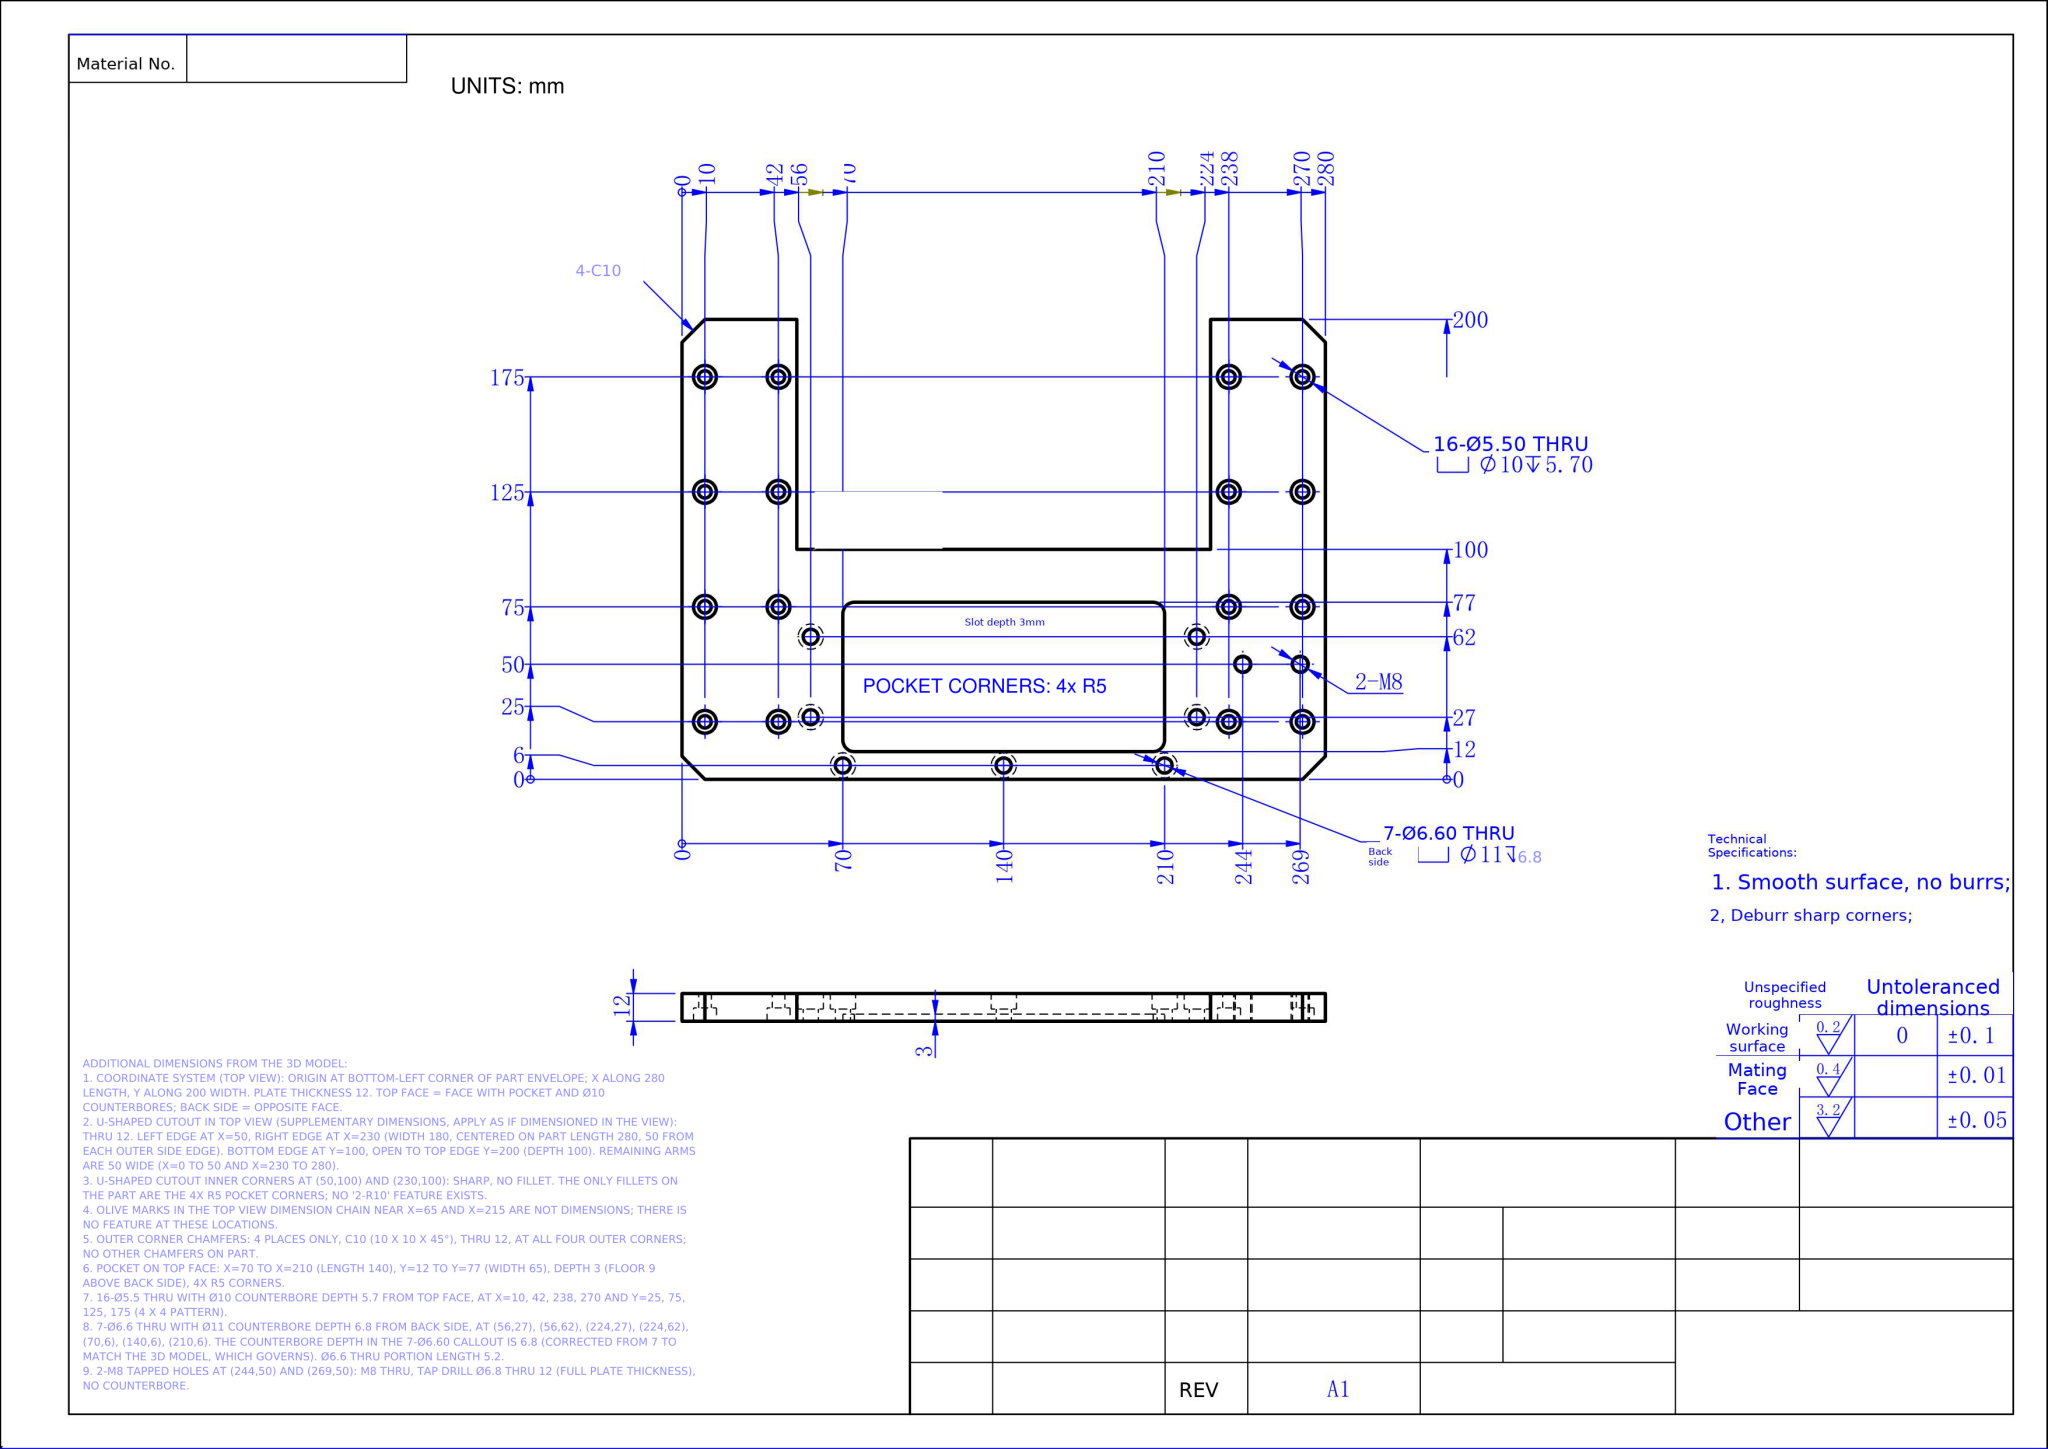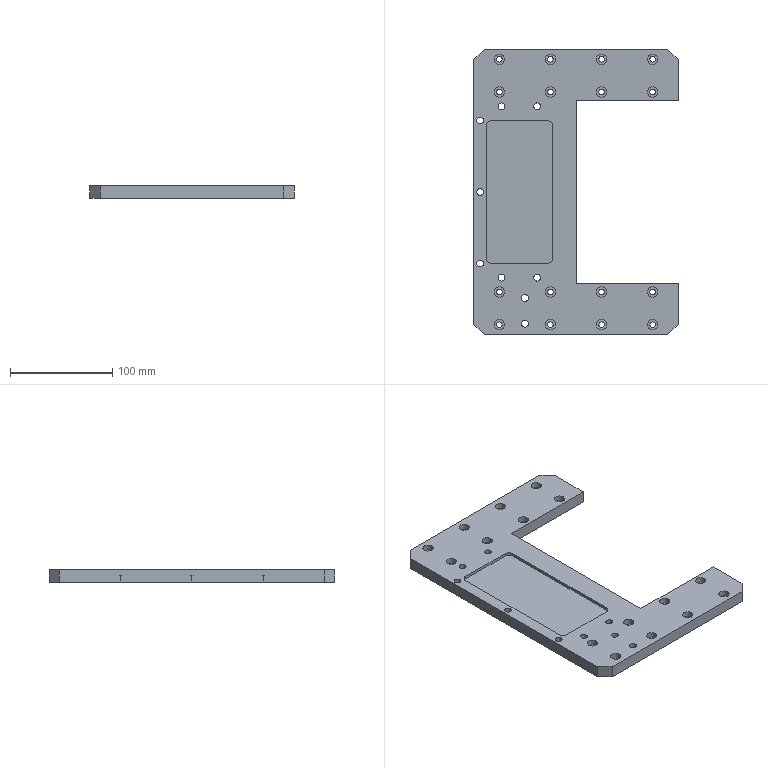Part | NX | mm | 1 solid | 142 faces | box 200 x 280 x 12 mm | volume 410166 mm3 | cylinder 100 | plane 42 | commonest cylinder face diameters 10 x36 5.5 x32 11 x14 6.6 x14 6.8 x4